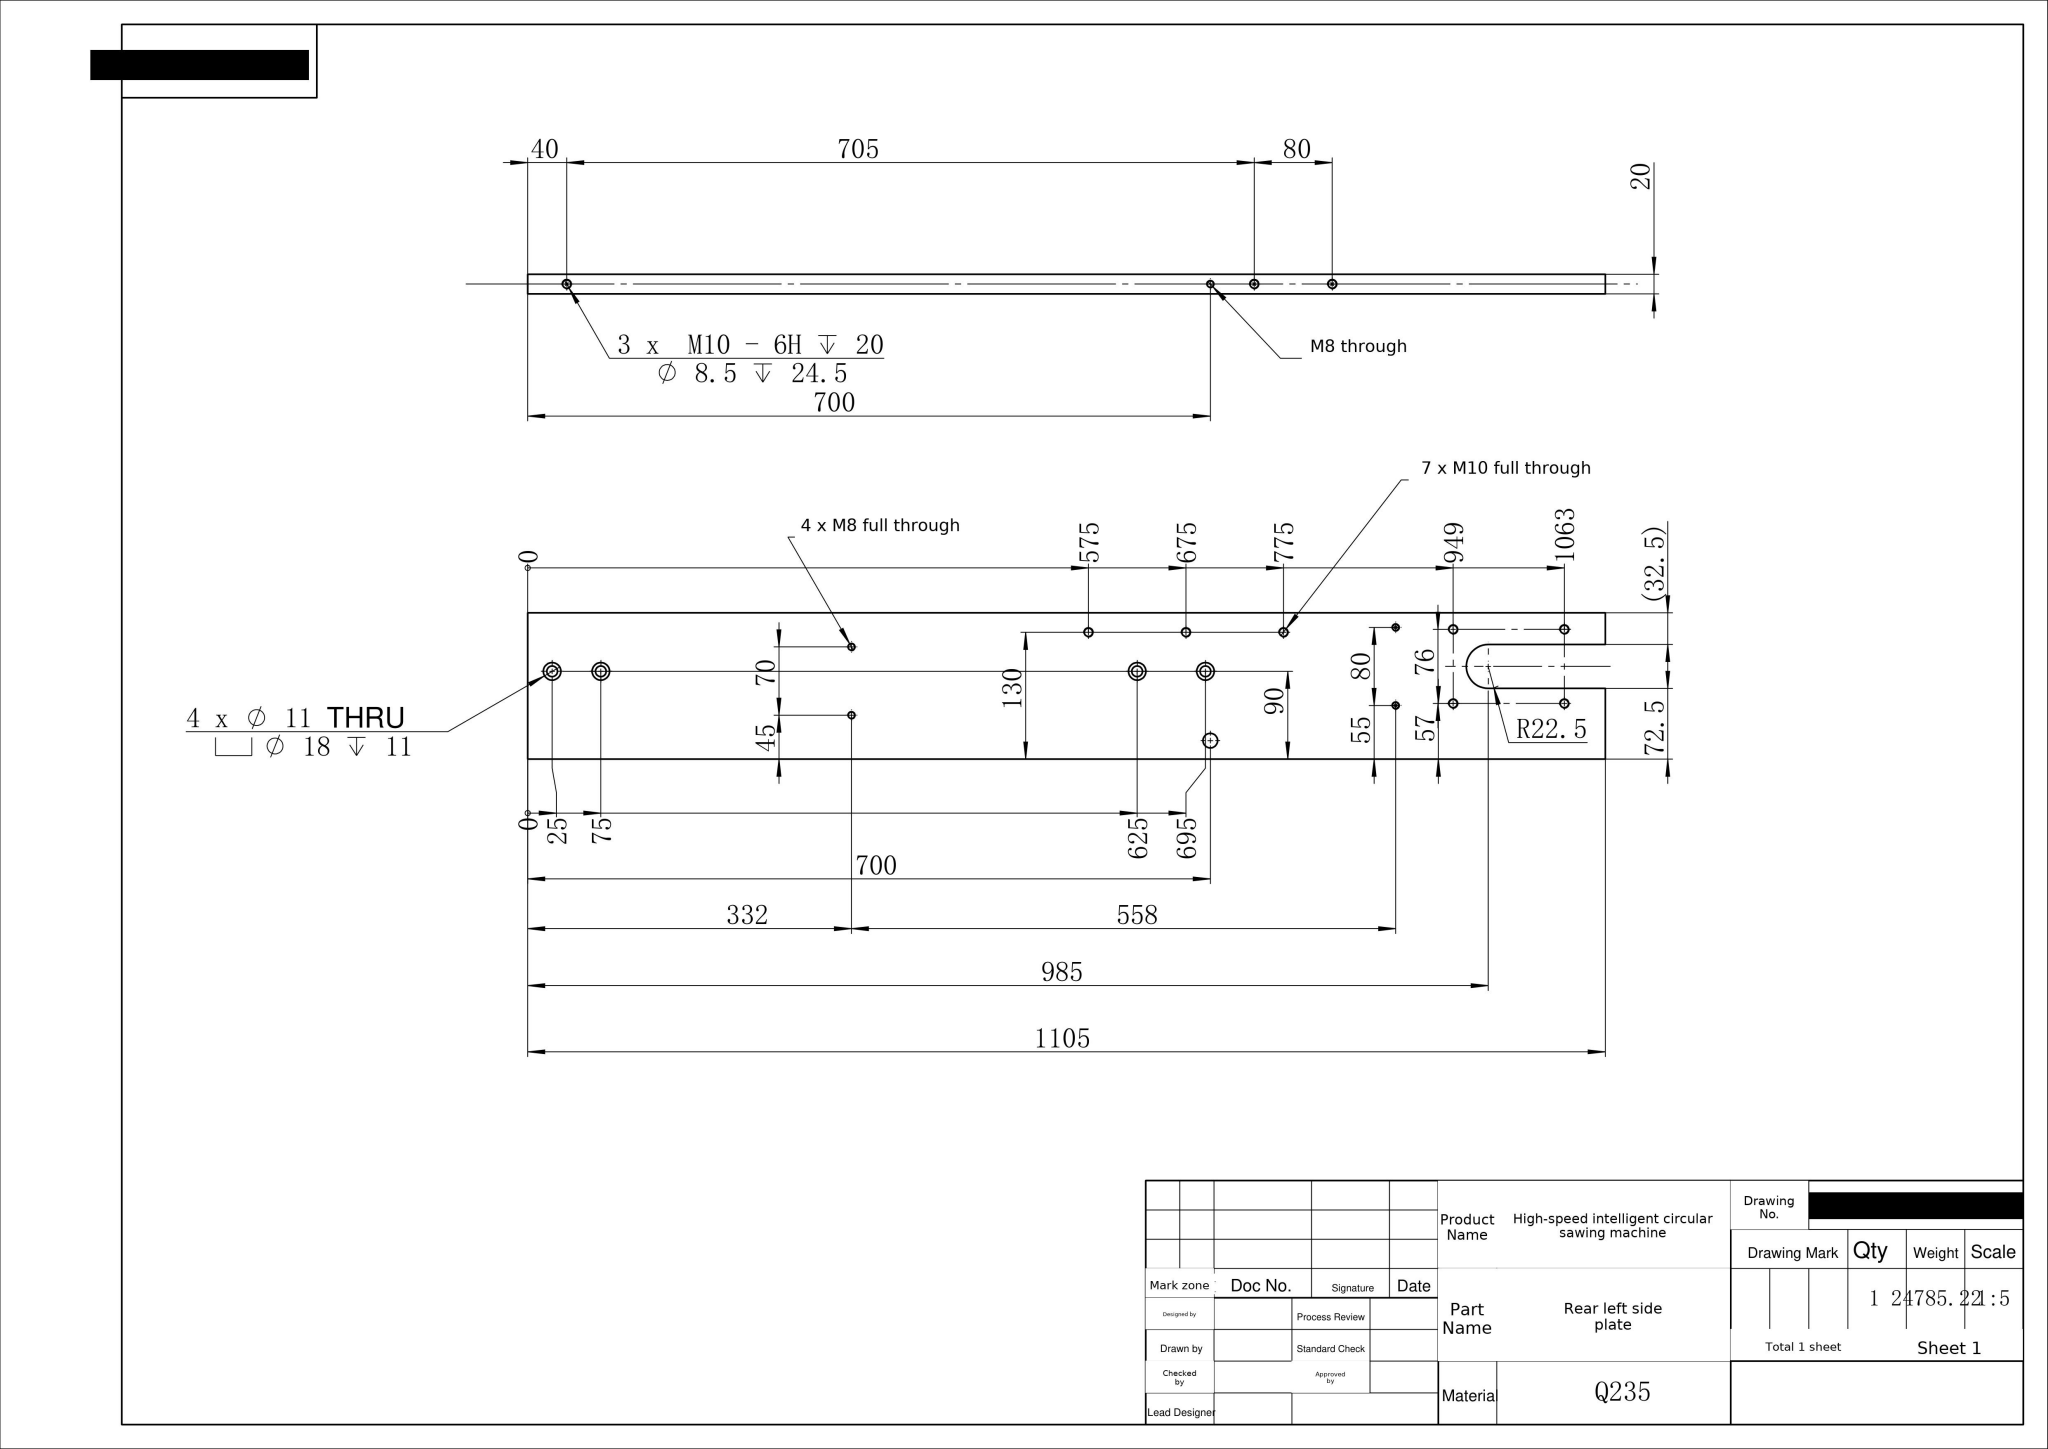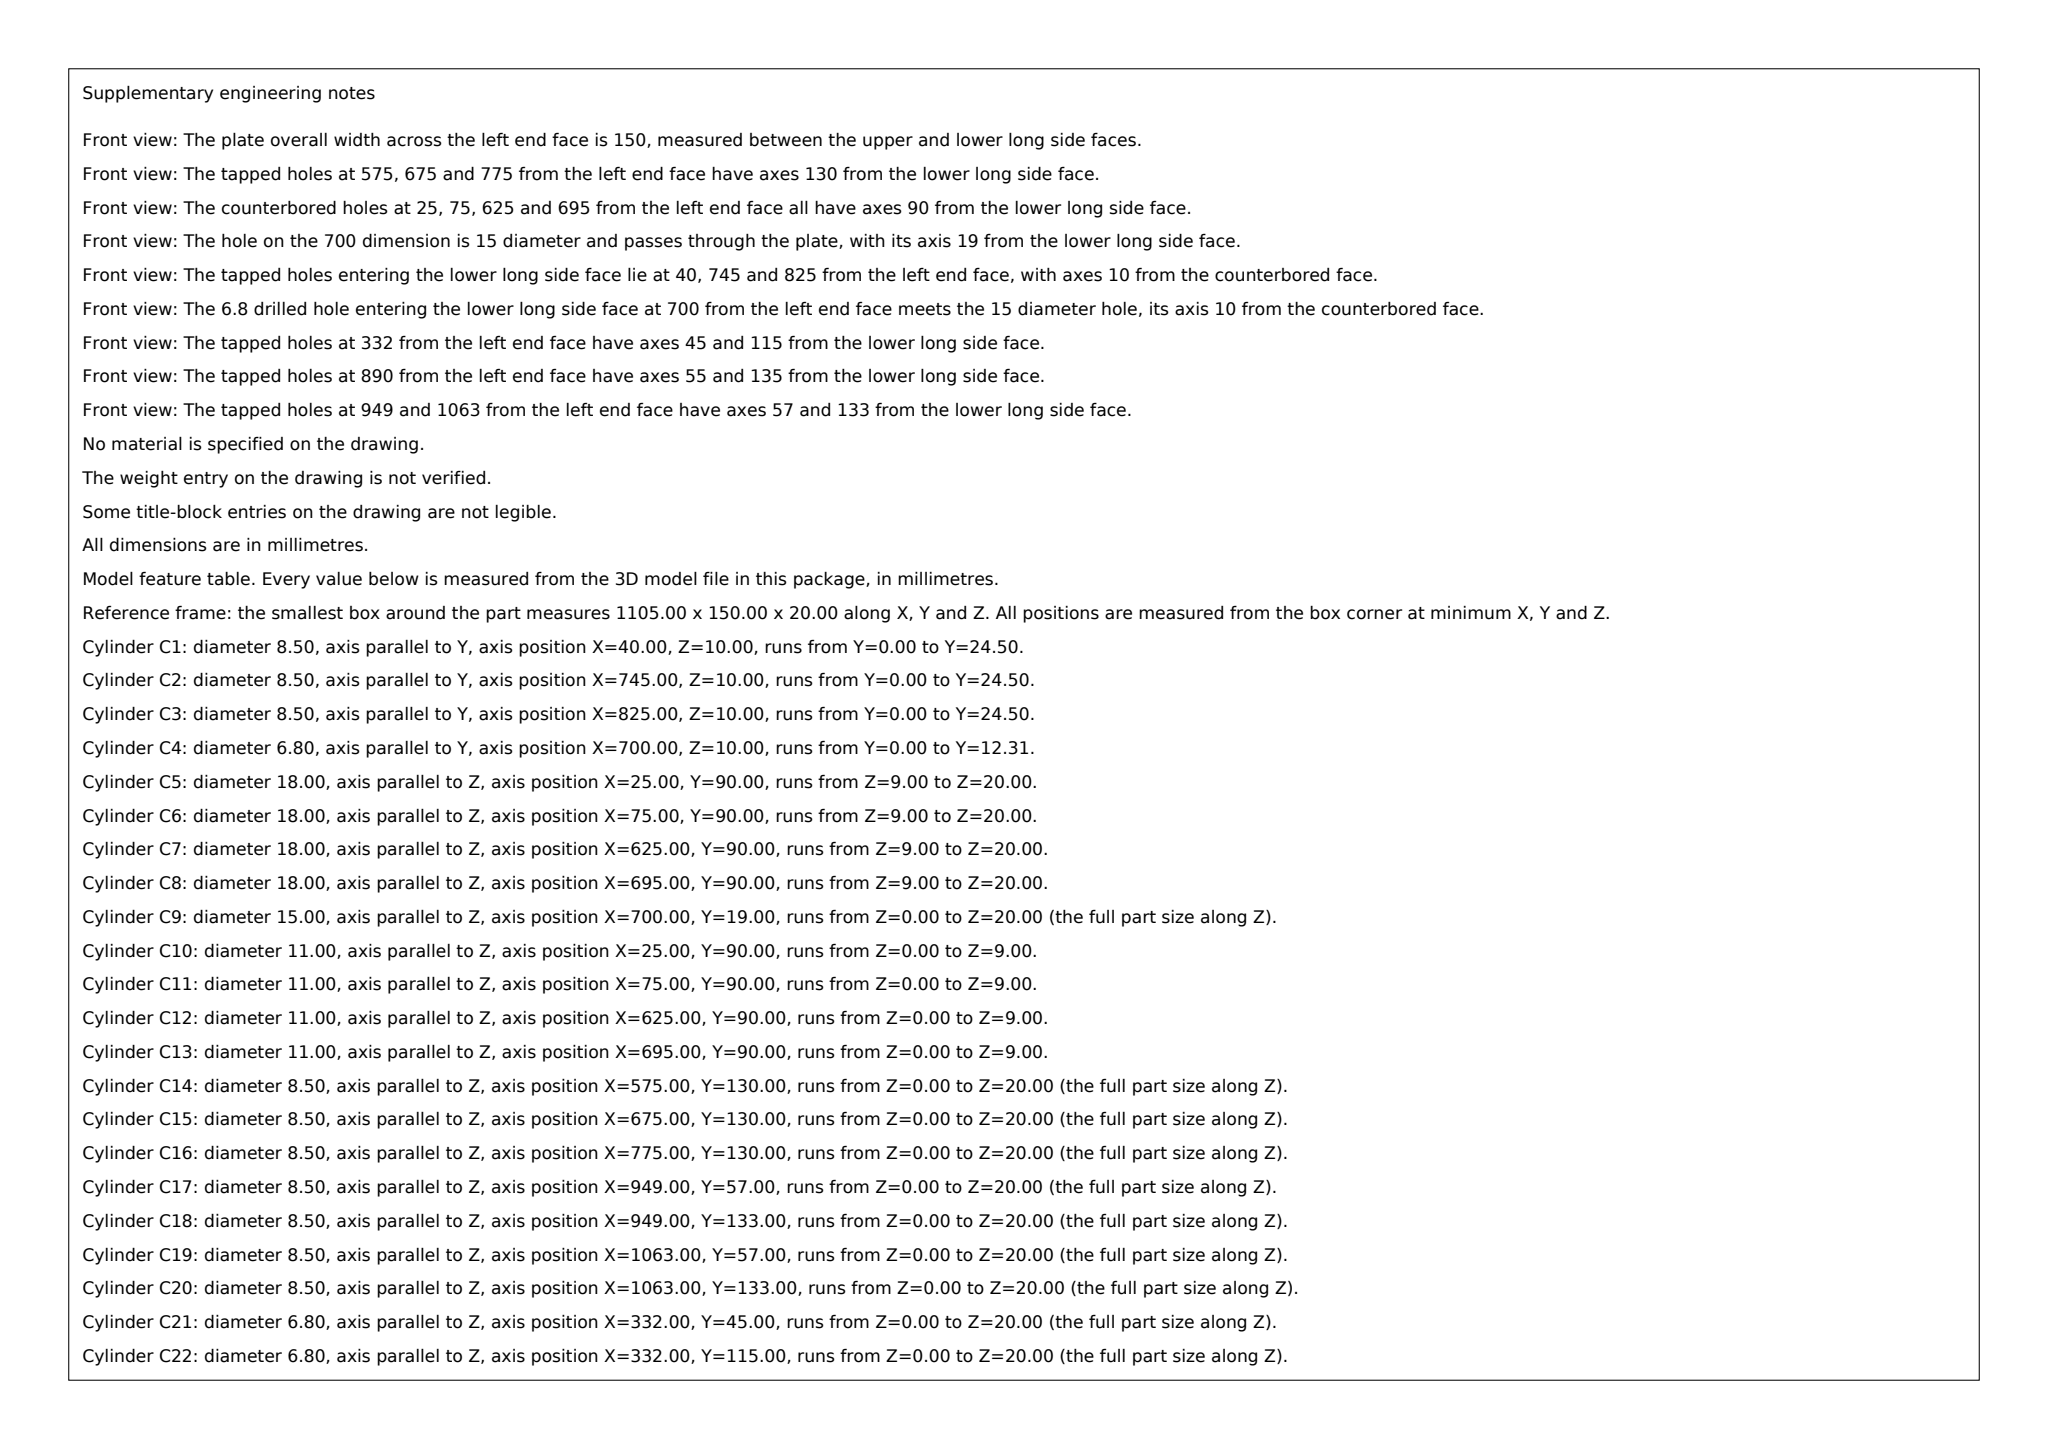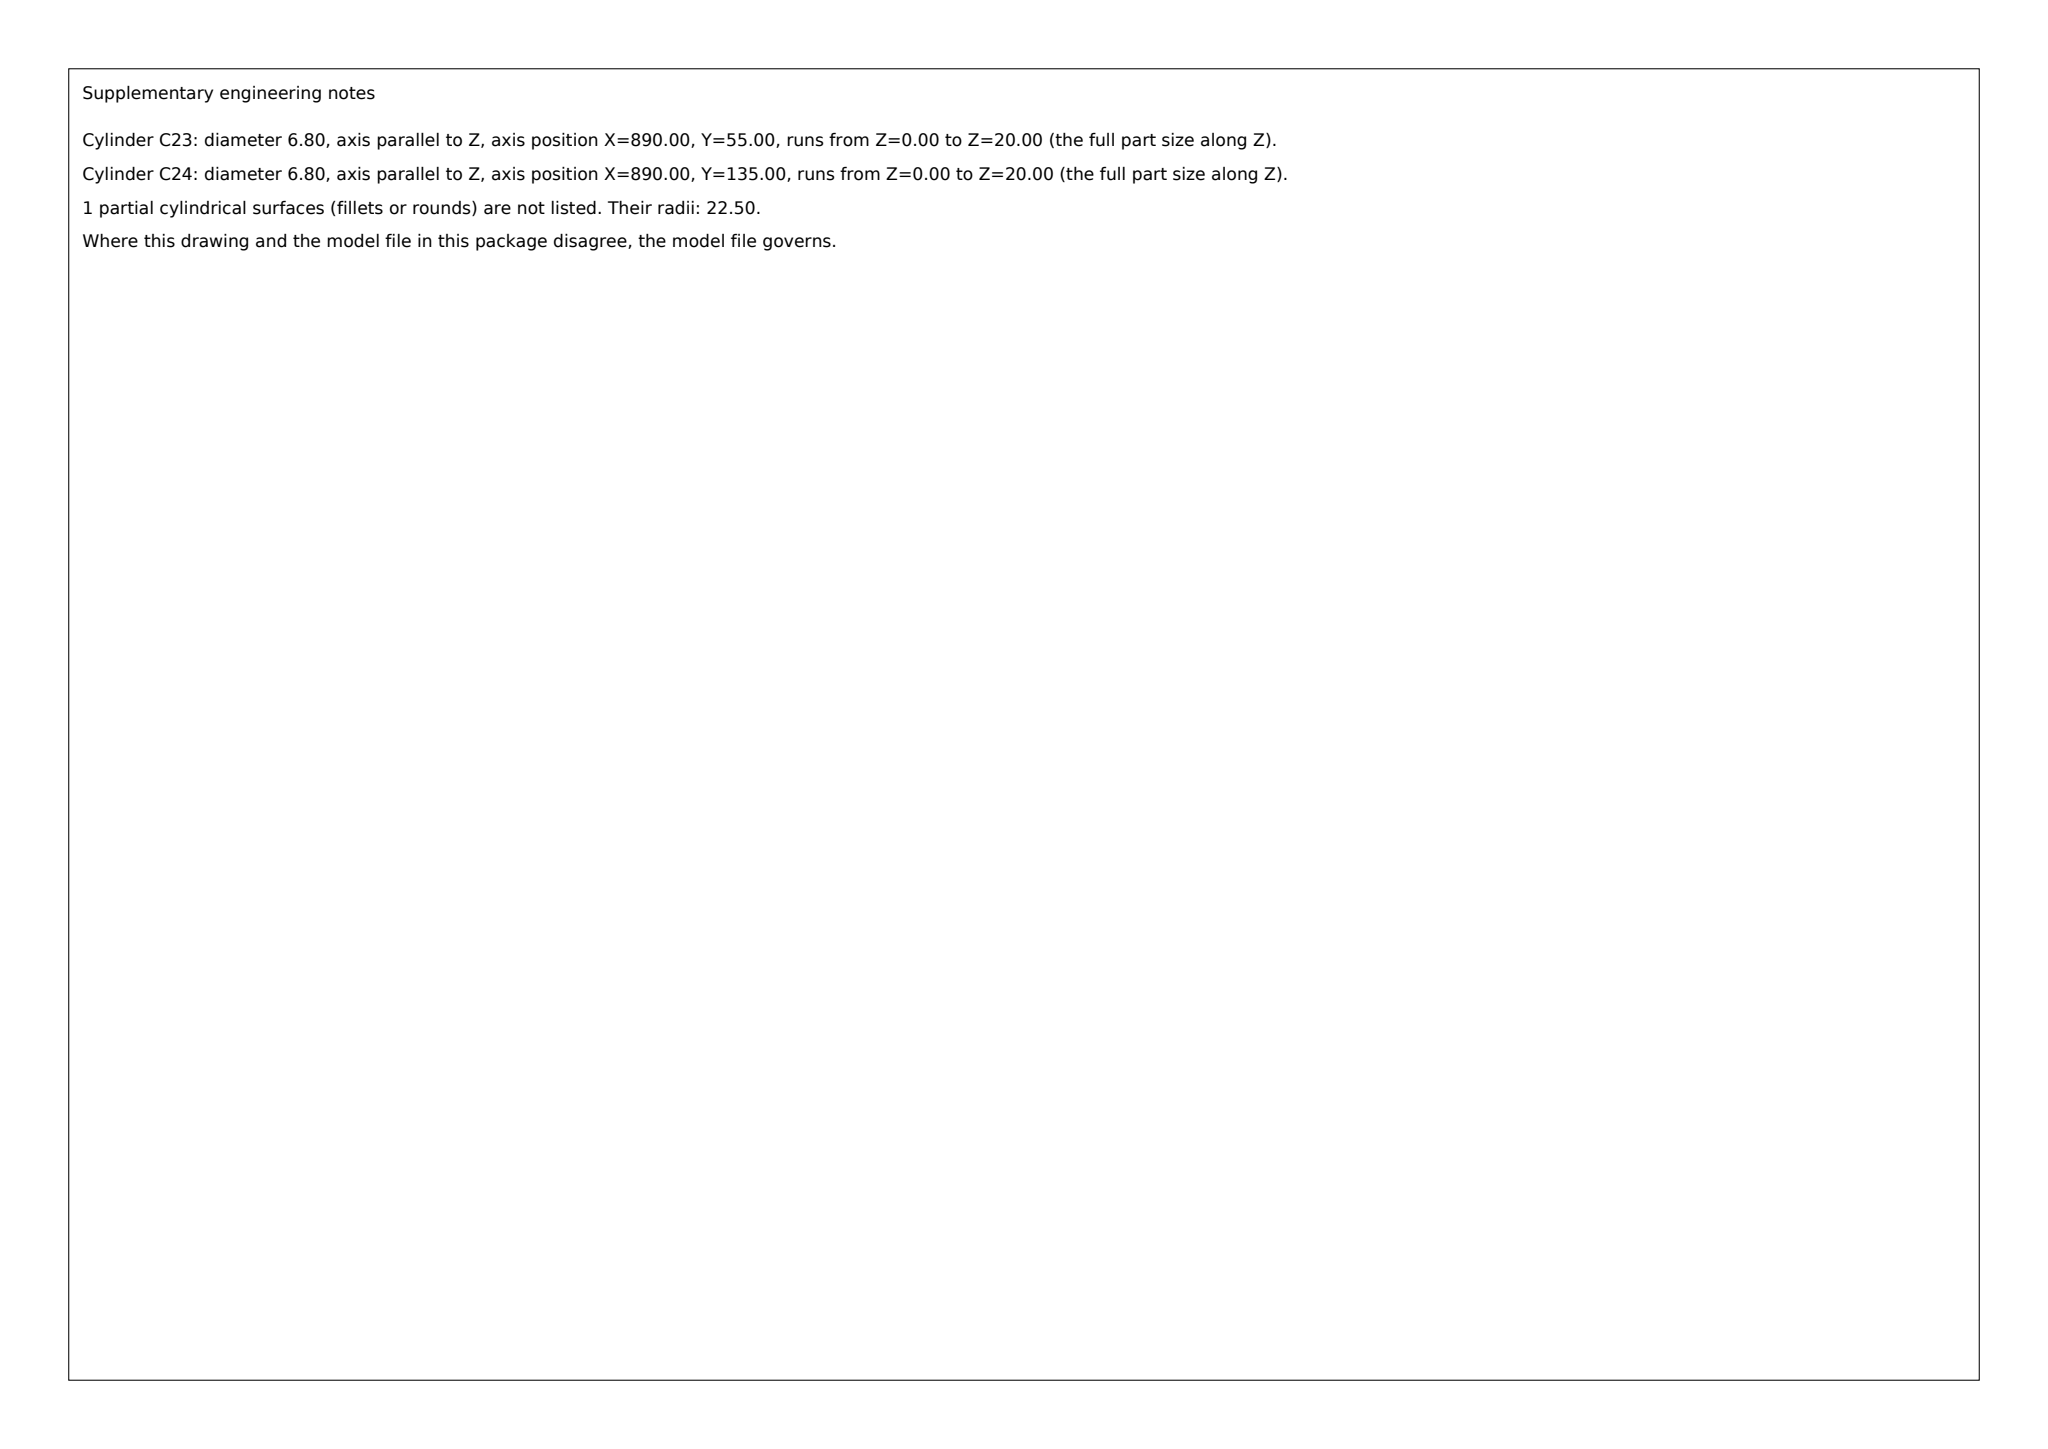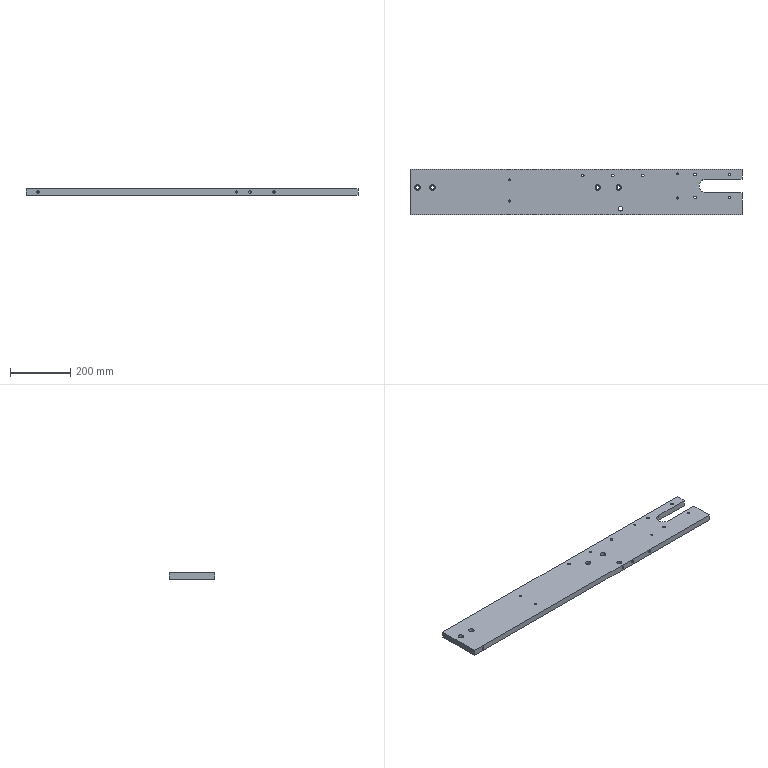Part | SolidWorks | mm | 1 solid | 68 faces | box 1105 x 150 x 20 mm | volume 3157353 mm3 | cylinder 49 | plane 13 | cone 6 | commonest cylinder face diameters 8.5 x20 6.8 x10 18 x8 11 x8 15 x2 45 x1
Drawing notes:
1X Ø15 THRU (20 THK), located X=700, Y=19 from lower-left corner of plate | from the solid: cylinder dia 15.0, axis z, pos [700.0, 19.0], length 20.0 = plate thickness (z planes at 0.0 and 20.0)
UNLESS OTHERWISE SPECIFIED, ALL DIMENSIONS ARE IN MILLIMETERS | from the solid: STEP model facts stated in mm
build123d program:
from build123d import *

# Parameters (mm, degrees)
SKETCH3_R                                          = 31
BOSS_EXTRUDE1_DEPTH                                = 20
HOLE_SIZE_ACCORDING_TO_TYPE_1_OF_HEXAG_D           = 11
HOLE_SIZE_ACCORDING_TO_TYPE_1_OF_HEXAG_CBORE_D     = 18
HOLE_SIZE_ACCORDING_TO_TYPE_1_OF_HEXAG_CBORE_DEPTH = 11
M8_TAPPED_HOLE1_D                                  = 6.8
SKETCH6_R                                          = 7.5
CUT_EXTRUDE1_DEPTH                                 = 1660.317
M8_TAPPED_HOLE2_REACH                              = 717.961
M8_TAPPED_HOLE2_BORE_R                             = 3.4
M10_TAPPED_HOLE1_D                                 = 8.5
M10_TAPPED_HOLE1_DEPTH                             = 24.5
M10_TAPPED_HOLE1_TIP                               = 2.554
SKETCH11_W                                         = 1105
SKETCH11_H                                         = 150
BOSS_EXTRUDE2_DEPTH                                = 20
HOLE_SIZE_ACCORDING_TO_TYPE_2_OF_H_2_COUNT         = 2
HOLE_SIZE_ACCORDING_TO_TYPE_2_OF_H_2_PITCH         = 50
HOLE_SIZE_ACCORDING_TO_TYPE_2_OF_H_3_COUNT         = 2
HOLE_SIZE_ACCORDING_TO_TYPE_2_OF_H_3_PITCH         = 492.5
HOLE_SIZE_ACCORDING_TO_TYPE_2_OF_H_4_COUNT         = 2
HOLE_SIZE_ACCORDING_TO_TYPE_2_OF_H_4_PITCH         = 562.5
HOLE_SIZE_ACCORDING_TO_TYPE_2_OF_H_5_COUNT         = 2
HOLE_SIZE_ACCORDING_TO_TYPE_2_OF_H_5_PITCH         = 1005
HOLE_SIZE_ACCORDING_TO_TYPE_2_OF_H_6_COUNT         = 2
HOLE_SIZE_ACCORDING_TO_TYPE_2_OF_H_6_PITCH         = 1055
SKETCH13_R                                         = 7.5
CUT_EXTRUDE2_DEPTH                                 = 1660.317
SKETCH15_W                                         = 3.4
SKETCH15_H                                         = 19
M8_TAPPED_HOLE3_AT_2_COUNT                         = 2
M8_TAPPED_HOLE3_AT_2_PITCH                         = 905
BOSS_EXTRUDE3_DEPTH                                = 20
HOLE_SIZE_ACCORDING_TO_TYPE_3_OF_H_2_COUNT         = 2
HOLE_SIZE_ACCORDING_TO_TYPE_3_OF_H_2_PITCH         = 50
HOLE_SIZE_ACCORDING_TO_TYPE_3_OF_H_3_COUNT         = 2
HOLE_SIZE_ACCORDING_TO_TYPE_3_OF_H_3_PITCH         = 670
HOLE_SIZE_ACCORDING_TO_TYPE_3_OF_H_4_COUNT         = 2
HOLE_SIZE_ACCORDING_TO_TYPE_3_OF_H_4_PITCH         = 600
SKETCH18_R                                         = 7.5
CUT_EXTRUDE3_DEPTH                                 = 1660.317
SKETCH20_W                                         = 3.4
SKETCH20_H                                         = 19
SKETCH21_W                                         = 4.25
SKETCH21_H                                         = 20
M10_TAPPED_HOLE2_AT_2_COUNT                        = 2
M10_TAPPED_HOLE2_AT_2_PITCH                        = 76
M10_TAPPED_HOLE2_AT_3_COUNT                        = 2
M10_TAPPED_HOLE2_AT_3_PITCH                        = 137.011
M10_TAPPED_HOLE2_AT_4_COUNT                        = 2
M10_TAPPED_HOLE2_AT_4_PITCH                        = 114
SKETCH23_W                                         = 3.4
SKETCH23_H                                         = 20
M8_TAPPED_HOLE5_AT_2_COUNT                         = 2
M8_TAPPED_HOLE5_AT_2_PITCH                         = 80
M10_TAPPED_HOLE3_AT_2_COUNT                        = 2
M10_TAPPED_HOLE3_AT_2_PITCH                        = 246
M10_TAPPED_HOLE3_AT_3_COUNT                        = 2
M10_TAPPED_HOLE3_AT_3_PITCH                        = 326
M10_TAPPED_HOLE4_AT_2_COUNT                        = 2
M10_TAPPED_HOLE4_AT_2_PITCH                        = 1025
M10_TAPPED_HOLE5_AT_2_COUNT                        = 2
M10_TAPPED_HOLE5_AT_2_PITCH                        = 705
M10_TAPPED_HOLE5_AT_3_COUNT                        = 2
M10_TAPPED_HOLE5_AT_3_PITCH                        = 785
SKETCH33_W                                         = 3.4
SKETCH33_H                                         = 20
M8_TAPPED_HOLE6_AT_2_COUNT                         = 2
M8_TAPPED_HOLE6_AT_2_PITCH                         = 70
SKETCH35_W                                         = 3.4
SKETCH35_H                                         = 20
M8_TAPPED_HOLE7_AT_2_COUNT                         = 2
M8_TAPPED_HOLE7_AT_2_PITCH                         = 70
M8_TAPPED_HOLE7_AT_3_COUNT                         = 2
M8_TAPPED_HOLE7_AT_3_PITCH                         = 500
M8_TAPPED_HOLE7_AT_4_COUNT                         = 2
M8_TAPPED_HOLE7_AT_4_PITCH                         = 504.876
SKETCH37_W                                         = 3.4
SKETCH37_H                                         = 20
M8_TAPPED_HOLE8_AT_2_COUNT                         = 2
M8_TAPPED_HOLE8_AT_2_PITCH                         = 70
SKETCH39_W                                         = 4.25
SKETCH39_H                                         = 20
M10_TAPPED_HOLE6_AT_2_COUNT                        = 2
M10_TAPPED_HOLE6_AT_2_PITCH                        = 305
M10_TAPPED_HOLE6_AT_3_COUNT                        = 2
M10_TAPPED_HOLE6_AT_3_PITCH                        = 610
SKETCH41_W                                         = 4.25
SKETCH41_H                                         = 20
M10_TAPPED_HOLE7_AT_2_COUNT                        = 2
M10_TAPPED_HOLE7_AT_2_PITCH                        = 100
M10_TAPPED_HOLE7_AT_3_COUNT                        = 2
M10_TAPPED_HOLE7_AT_3_PITCH                        = 200
SKETCH42_W                                         = 2254.677
SKETCH42_H                                         = 350.493
CUT_EXTRUDE4_DEPTH                                 = 1660.317


with BuildPart() as part:
    # Sketch3 → Boss-Extrude1 (new body)
    with BuildSketch(Plane.XY):
        Polygon((-552.5, 75), (-552.5, -75), (-1657.5, -75), (-1657.5, 50), (-1614.199, 75), align=None)
        with Locations((-1582.5, 20)):
            Circle(SKETCH3_R, mode=Mode.SUBTRACT)
    extrude(amount=-BOSS_EXTRUDE1_DEPTH)

    # Hole Size _according to_ Type 1 of Hexag (through all)
    with Locations(Plane(origin=(-1297.5, 15, 0), x_dir=(1, 0, 0), z_dir=(0, 0, 1))):
        with Locations((0, 0), (70, 0), (670, 0), (720, 0)):
            CounterBoreHole(HOLE_SIZE_ACCORDING_TO_TYPE_1_OF_HEXAG_D / 2, HOLE_SIZE_ACCORDING_TO_TYPE_1_OF_HEXAG_CBORE_D / 2, HOLE_SIZE_ACCORDING_TO_TYPE_1_OF_HEXAG_CBORE_DEPTH)

    # M8 Tapped Hole1 (through all)
    with Locations(Plane(origin=(-1620.5, 20, 0), x_dir=(1, 0, 0), z_dir=(0, 0, 1))):
        with Locations((0, 0), (38, -38), (76, 0), (38, 38)):
            Hole(M8_TAPPED_HOLE1_D / 2)

    # Sketch6 → Cut-Extrude1 (cut, through all)
    with BuildSketch(Plane.XY):
        with Locations((-1252.5, -56)):
            Circle(SKETCH6_R)
    extrude(amount=-CUT_EXTRUDE1_DEPTH, mode=Mode.SUBTRACT)

    # M8 Tapped Hole2 bore (on position points) → M8 Tapped Hole2 (cut, up to next)
    with BuildSketch(Plane(origin=(-1252.5, -75, -10), x_dir=(0, 0, -1), z_dir=(0, -1, 0)), mode=Mode.PRIVATE) as m8_tapped_hole2_sk1:
        Circle(M8_TAPPED_HOLE2_BORE_R)
    m8_tapped_hole2_tool1 = extrude(m8_tapped_hole2_sk1.sketch, amount=-M8_TAPPED_HOLE2_REACH, mode=Mode.PRIVATE) & part.part
    add(m8_tapped_hole2_tool1.solids().sort_by_distance((-1252.5, -75, -10))[0], mode=Mode.SUBTRACT)

    # M10 Tapped Hole1
    with Locations(Plane(origin=(-1657.5, -5, -10), x_dir=(0, 0, -1), z_dir=(-1, 0, 0))):
        with Locations((0, 0), (0, 50)):
            Hole(M10_TAPPED_HOLE1_D / 2, depth=M10_TAPPED_HOLE1_DEPTH)
            with Locations((0, 0, -(M10_TAPPED_HOLE1_DEPTH + M10_TAPPED_HOLE1_TIP / 2))):  # 118° drill point
                Cone(0, M10_TAPPED_HOLE1_D / 2, M10_TAPPED_HOLE1_TIP, mode=Mode.SUBTRACT)

    # Sketch25 → M10 Tapped Hole3 (revolve, cut)
    with BuildSketch(Plane(origin=(-592.5, -75, -10), x_dir=(0, 0, -1), z_dir=(1, 0, 0))):
        Polygon((0, 0), (0, 27.054), (4.25, 24.5), (4.25, 0), align=None)
    m10_tapped_hole3 = revolve(axis=Axis((-592.5, -81.35, -10), (0, 1, 0)), mode=Mode.SUBTRACT)

    # M10 Tapped Hole3 at 2: M10 Tapped Hole3 ×2
    with Locations(*[(-i * M10_TAPPED_HOLE3_AT_2_PITCH, 0, 0) for i in range(1, M10_TAPPED_HOLE3_AT_2_COUNT)]):
        add(m10_tapped_hole3, mode=Mode.SUBTRACT)

    # M10 Tapped Hole3 at 3: M10 Tapped Hole3 ×2
    with Locations(*[(-i * M10_TAPPED_HOLE3_AT_3_PITCH, 0, 0) for i in range(1, M10_TAPPED_HOLE3_AT_3_COUNT)]):
        add(m10_tapped_hole3, mode=Mode.SUBTRACT)

    # Sketch33 → M8 Tapped Hole6 (revolve, cut)
    with BuildSketch(Plane(origin=(-595.5, 40, 0), x_dir=(0, -1, 0), z_dir=(1, 0, 0))):
        with Locations((1.7, 10)):
            Rectangle(SKETCH33_W, SKETCH33_H)
    m8_tapped_hole6 = revolve(axis=Axis((-595.5, 40, 6.35), (0, 0, -1)), mode=Mode.SUBTRACT)

    # M8 Tapped Hole6 at 2: M8 Tapped Hole6 ×2
    with Locations(*[(0, -i * M8_TAPPED_HOLE6_AT_2_PITCH, 0) for i in range(1, M8_TAPPED_HOLE6_AT_2_COUNT)]):
        add(m8_tapped_hole6, mode=Mode.SUBTRACT)

    # Sketch39 → M10 Tapped Hole6 (revolve, cut)
    with BuildSketch(Plane(origin=(-1511.5, 55, 0), x_dir=(0, -1, 0), z_dir=(1, 0, 0))):
        with Locations((2.125, 10)):
            Rectangle(SKETCH39_W, SKETCH39_H)
    m10_tapped_hole6 = revolve(axis=Axis((-1511.5, 55, 6.35), (0, 0, -1)), mode=Mode.SUBTRACT)

    # M10 Tapped Hole6 at 2: M10 Tapped Hole6 ×2
    with Locations(*[(i * M10_TAPPED_HOLE6_AT_2_PITCH, 0, 0) for i in range(1, M10_TAPPED_HOLE6_AT_2_COUNT)]):
        add(m10_tapped_hole6, mode=Mode.SUBTRACT)

    # M10 Tapped Hole6 at 3: M10 Tapped Hole6 ×2
    with Locations(*[(i * M10_TAPPED_HOLE6_AT_3_PITCH, 0, 0) for i in range(1, M10_TAPPED_HOLE6_AT_3_COUNT)]):
        add(m10_tapped_hole6, mode=Mode.SUBTRACT)


with BuildPart() as body_2:
    # Sketch11 → Boss-Extrude2 (new body)
    with BuildSketch(Plane.XY):
        Rectangle(SKETCH11_W, SKETCH11_H)
    extrude(amount=-BOSS_EXTRUDE2_DEPTH)

    # Sketch12 → Hole Size _according to_ Type 2 of Hexag (revolve, cut)
    with BuildSketch(Plane(origin=(-527.5, 15, 0), x_dir=(0, -1, 0), z_dir=(1, 0, 0))):
        Polygon((0, 0), (0, 20), (5.5, 20), (5.5, 11), (9, 11), (9, 0), align=None)
    hole_size_according_to_type_2_of_hexag = revolve(axis=Axis((-527.5, 15, 6.35), (0, 0, -1)), mode=Mode.SUBTRACT)

    # Hole Size _according to_ Type 2 of H 2: Hole Size _according to_ Type 2 of Hexag ×2
    with Locations(*[(i * HOLE_SIZE_ACCORDING_TO_TYPE_2_OF_H_2_PITCH, 0, 0) for i in range(1, HOLE_SIZE_ACCORDING_TO_TYPE_2_OF_H_2_COUNT)]):
        add(hole_size_according_to_type_2_of_hexag, mode=Mode.SUBTRACT)

    # Hole Size _according to_ Type 2 of H 3: Hole Size _according to_ Type 2 of Hexag ×2
    with Locations(*[(i * HOLE_SIZE_ACCORDING_TO_TYPE_2_OF_H_3_PITCH, 0, 0) for i in range(1, HOLE_SIZE_ACCORDING_TO_TYPE_2_OF_H_3_COUNT)]):
        add(hole_size_according_to_type_2_of_hexag, mode=Mode.SUBTRACT)

    # Hole Size _according to_ Type 2 of H 4: Hole Size _according to_ Type 2 of Hexag ×2
    with Locations(*[(i * HOLE_SIZE_ACCORDING_TO_TYPE_2_OF_H_4_PITCH, 0, 0) for i in range(1, HOLE_SIZE_ACCORDING_TO_TYPE_2_OF_H_4_COUNT)]):
        add(hole_size_according_to_type_2_of_hexag, mode=Mode.SUBTRACT)

    # Hole Size _according to_ Type 2 of H 5: Hole Size _according to_ Type 2 of Hexag ×2
    with Locations(*[(i * HOLE_SIZE_ACCORDING_TO_TYPE_2_OF_H_5_PITCH, 0, 0) for i in range(1, HOLE_SIZE_ACCORDING_TO_TYPE_2_OF_H_5_COUNT)]):
        add(hole_size_according_to_type_2_of_hexag, mode=Mode.SUBTRACT)

    # Hole Size _according to_ Type 2 of H 6: Hole Size _according to_ Type 2 of Hexag ×2
    with Locations(*[(i * HOLE_SIZE_ACCORDING_TO_TYPE_2_OF_H_6_PITCH, 0, 0) for i in range(1, HOLE_SIZE_ACCORDING_TO_TYPE_2_OF_H_6_COUNT)]):
        add(hole_size_according_to_type_2_of_hexag, mode=Mode.SUBTRACT)

    # Sketch13 → Cut-Extrude2 (cut, through all)
    with BuildSketch(Plane.XY):
        with Locations((452.5, -56)):
            Circle(SKETCH13_R)
        with Locations((-452.5, -56)):
            Circle(SKETCH13_R)
    extrude(amount=-CUT_EXTRUDE2_DEPTH, mode=Mode.SUBTRACT)

    # Sketch15 → M8 Tapped Hole3 (revolve, cut)
    with BuildSketch(Plane(origin=(-452.5, -75, -10), x_dir=(0, 0, -1), z_dir=(1, 0, 0))):
        with Locations((1.7, 9.5)):
            Rectangle(SKETCH15_W, SKETCH15_H)
    m8_tapped_hole3 = revolve(axis=Axis((-452.5, -81.35, -10), (0, 1, 0)), mode=Mode.SUBTRACT)

    # M8 Tapped Hole3 at 2: M8 Tapped Hole3 ×2
    with Locations(*[(i * M8_TAPPED_HOLE3_AT_2_PITCH, 0, 0) for i in range(1, M8_TAPPED_HOLE3_AT_2_COUNT)]):
        add(m8_tapped_hole3, mode=Mode.SUBTRACT)

    # Sketch27 → M10 Tapped Hole4 (revolve, cut)
    with BuildSketch(Plane(origin=(-512.5, -75, -10), x_dir=(0, 0, -1), z_dir=(1, 0, 0))):
        Polygon((0, 0), (0, 27.054), (4.25, 24.5), (4.25, 0), align=None)
    m10_tapped_hole4 = revolve(axis=Axis((-512.5, -81.35, -10), (0, 1, 0)), mode=Mode.SUBTRACT)

    # M10 Tapped Hole4 at 2: M10 Tapped Hole4 ×2
    with Locations(*[(i * M10_TAPPED_HOLE4_AT_2_PITCH, 0, 0) for i in range(1, M10_TAPPED_HOLE4_AT_2_COUNT)]):
        add(m10_tapped_hole4, mode=Mode.SUBTRACT)

    # Sketch35 → M8 Tapped Hole7 (revolve, cut)
    with BuildSketch(Plane(origin=(-105.5, 40, 0), x_dir=(0, -1, 0), z_dir=(1, 0, 0))):
        with Locations((1.7, 10)):
            Rectangle(SKETCH35_W, SKETCH35_H)
    m8_tapped_hole7 = revolve(axis=Axis((-105.5, 40, 6.35), (0, 0, -1)), mode=Mode.SUBTRACT)

    # M8 Tapped Hole7 at 2: M8 Tapped Hole7 ×2
    with Locations(*[(0, -i * M8_TAPPED_HOLE7_AT_2_PITCH, 0) for i in range(1, M8_TAPPED_HOLE7_AT_2_COUNT)]):
        add(m8_tapped_hole7, mode=Mode.SUBTRACT)

    # M8 Tapped Hole7 at 3: M8 Tapped Hole7 ×2
    with Locations(*[(i * M8_TAPPED_HOLE7_AT_3_PITCH, 0, 0) for i in range(1, M8_TAPPED_HOLE7_AT_3_COUNT)]):
        add(m8_tapped_hole7, mode=Mode.SUBTRACT)

    # M8 Tapped Hole7 at 4: M8 Tapped Hole7 ×2
    with Locations(*[Vector(0.9903, -0.1386, 0) * (i * M8_TAPPED_HOLE7_AT_4_PITCH) for i in range(1, M8_TAPPED_HOLE7_AT_4_COUNT)]):
        add(m8_tapped_hole7, mode=Mode.SUBTRACT)


with BuildPart() as body_3:
    # Sketch16 → Boss-Extrude3 (new body)
    with BuildSketch(Plane.XY):
        with BuildLine():
            Line((552.5, 75), (1657.5, 75))
            Line((1657.5, 75), (1657.5, 42.5))
            Line((1657.5, 42.5), (1537.5, 42.5))
            ThreePointArc((1537.5, 42.5), (1515, 20), (1537.5, -2.5))
            Line((1537.5, -2.5), (1657.5, -2.5))
            Line((1657.5, -2.5), (1657.5, -75))
            Line((1657.5, -75), (552.5, -75))
            Line((552.5, -75), (552.5, 75))
        make_face()
    extrude(amount=-BOSS_EXTRUDE3_DEPTH)

    # Sketch17 → Hole Size _according to_ Type 3 of Hexag (revolve, cut)
    with BuildSketch(Plane(origin=(577.5, 15, 0), x_dir=(0, -1, 0), z_dir=(1, 0, 0))):
        Polygon((0, 0), (0, 20), (5.5, 20), (5.5, 11), (9, 11), (9, 0), align=None)
    hole_size_according_to_type_3_of_hexag = revolve(axis=Axis((577.5, 15, 6.35), (0, 0, -1)), mode=Mode.SUBTRACT)

    # Hole Size _according to_ Type 3 of H 2: Hole Size _according to_ Type 3 of Hexag ×2
    with Locations(*[(i * HOLE_SIZE_ACCORDING_TO_TYPE_3_OF_H_2_PITCH, 0, 0) for i in range(1, HOLE_SIZE_ACCORDING_TO_TYPE_3_OF_H_2_COUNT)]):
        add(hole_size_according_to_type_3_of_hexag, mode=Mode.SUBTRACT)

    # Hole Size _according to_ Type 3 of H 3: Hole Size _according to_ Type 3 of Hexag ×2
    with Locations(*[(i * HOLE_SIZE_ACCORDING_TO_TYPE_3_OF_H_3_PITCH, 0, 0) for i in range(1, HOLE_SIZE_ACCORDING_TO_TYPE_3_OF_H_3_COUNT)]):
        add(hole_size_according_to_type_3_of_hexag, mode=Mode.SUBTRACT)

    # Hole Size _according to_ Type 3 of H 4: Hole Size _according to_ Type 3 of Hexag ×2
    with Locations(*[(i * HOLE_SIZE_ACCORDING_TO_TYPE_3_OF_H_4_PITCH, 0, 0) for i in range(1, HOLE_SIZE_ACCORDING_TO_TYPE_3_OF_H_4_COUNT)]):
        add(hole_size_according_to_type_3_of_hexag, mode=Mode.SUBTRACT)

    # Sketch18 → Cut-Extrude3 (cut, through all)
    with BuildSketch(Plane.XY):
        with Locations((1252.5, -56)):
            Circle(SKETCH18_R)
    extrude(amount=-CUT_EXTRUDE3_DEPTH, mode=Mode.SUBTRACT)

    # Sketch20 → M8 Tapped Hole4 (revolve, cut)
    with BuildSketch(Plane(origin=(1252.5, -75, -10), x_dir=(0, 0, -1), z_dir=(1, 0, 0))):
        with Locations((1.7, 9.5)):
            Rectangle(SKETCH20_W, SKETCH20_H)
    revolve(axis=Axis((1252.5, -81.35, -10), (0, 1, 0)), mode=Mode.SUBTRACT)

    # Sketch21 → M10 Tapped Hole2 (revolve, cut)
    with BuildSketch(Plane(origin=(1501.5, 58, 0), x_dir=(0, -1, 0), z_dir=(1, 0, 0))):
        with Locations((2.125, 10)):
            Rectangle(SKETCH21_W, SKETCH21_H)
    m10_tapped_hole2 = revolve(axis=Axis((1501.5, 58, 6.35), (0, 0, -1)), mode=Mode.SUBTRACT)

    # M10 Tapped Hole2 at 2: M10 Tapped Hole2 ×2
    with Locations(*[(0, -i * M10_TAPPED_HOLE2_AT_2_PITCH, 0) for i in range(1, M10_TAPPED_HOLE2_AT_2_COUNT)]):
        add(m10_tapped_hole2, mode=Mode.SUBTRACT)

    # M10 Tapped Hole2 at 3: M10 Tapped Hole2 ×2
    with Locations(*[Vector(0.8321, -0.5547, 0) * (i * M10_TAPPED_HOLE2_AT_3_PITCH) for i in range(1, M10_TAPPED_HOLE2_AT_3_COUNT)]):
        add(m10_tapped_hole2, mode=Mode.SUBTRACT)

    # M10 Tapped Hole2 at 4: M10 Tapped Hole2 ×2
    with Locations(*[(i * M10_TAPPED_HOLE2_AT_4_PITCH, 0, 0) for i in range(1, M10_TAPPED_HOLE2_AT_4_COUNT)]):
        add(m10_tapped_hole2, mode=Mode.SUBTRACT)

    # Sketch23 → M8 Tapped Hole5 (revolve, cut)
    with BuildSketch(Plane(origin=(1442.5, 60, 0), x_dir=(0, -1, 0), z_dir=(1, 0, 0))):
        with Locations((1.7, 10)):
            Rectangle(SKETCH23_W, SKETCH23_H)
    m8_tapped_hole5 = revolve(axis=Axis((1442.5, 60, 6.35), (0, 0, -1)), mode=Mode.SUBTRACT)

    # M8 Tapped Hole5 at 2: M8 Tapped Hole5 ×2
    with Locations(*[(0, -i * M8_TAPPED_HOLE5_AT_2_PITCH, 0) for i in range(1, M8_TAPPED_HOLE5_AT_2_COUNT)]):
        add(m8_tapped_hole5, mode=Mode.SUBTRACT)

    # Sketch31 → M10 Tapped Hole5 (revolve, cut)
    with BuildSketch(Plane(origin=(592.5, -75, -10), x_dir=(0, 0, -1), z_dir=(1, 0, 0))):
        Polygon((0, 0), (0, 27.054), (4.25, 24.5), (4.25, 0), align=None)
    m10_tapped_hole5 = revolve(axis=Axis((592.5, -81.35, -10), (0, 1, 0)), mode=Mode.SUBTRACT)

    # M10 Tapped Hole5 at 2: M10 Tapped Hole5 ×2
    with Locations(*[(i * M10_TAPPED_HOLE5_AT_2_PITCH, 0, 0) for i in range(1, M10_TAPPED_HOLE5_AT_2_COUNT)]):
        add(m10_tapped_hole5, mode=Mode.SUBTRACT)

    # M10 Tapped Hole5 at 3: M10 Tapped Hole5 ×2
    with Locations(*[(i * M10_TAPPED_HOLE5_AT_3_PITCH, 0, 0) for i in range(1, M10_TAPPED_HOLE5_AT_3_COUNT)]):
        add(m10_tapped_hole5, mode=Mode.SUBTRACT)

    # Sketch37 → M8 Tapped Hole8 (revolve, cut)
    with BuildSketch(Plane(origin=(884.5, 40, 0), x_dir=(0, -1, 0), z_dir=(1, 0, 0))):
        with Locations((1.7, 10)):
            Rectangle(SKETCH37_W, SKETCH37_H)
    m8_tapped_hole8 = revolve(axis=Axis((884.5, 40, 6.35), (0, 0, -1)), mode=Mode.SUBTRACT)

    # M8 Tapped Hole8 at 2: M8 Tapped Hole8 ×2
    with Locations(*[(0, -i * M8_TAPPED_HOLE8_AT_2_PITCH, 0) for i in range(1, M8_TAPPED_HOLE8_AT_2_COUNT)]):
        add(m8_tapped_hole8, mode=Mode.SUBTRACT)

    # Sketch41 → M10 Tapped Hole7 (revolve, cut)
    with BuildSketch(Plane(origin=(1127.5, 55, 0), x_dir=(0, -1, 0), z_dir=(1, 0, 0))):
        with Locations((2.125, 10)):
            Rectangle(SKETCH41_W, SKETCH41_H)
    m10_tapped_hole7 = revolve(axis=Axis((1127.5, 55, 6.35), (0, 0, -1)), mode=Mode.SUBTRACT)

    # M10 Tapped Hole7 at 2: M10 Tapped Hole7 ×2
    with Locations(*[(i * M10_TAPPED_HOLE7_AT_2_PITCH, 0, 0) for i in range(1, M10_TAPPED_HOLE7_AT_2_COUNT)]):
        add(m10_tapped_hole7, mode=Mode.SUBTRACT)

    # M10 Tapped Hole7 at 3: M10 Tapped Hole7 ×2
    with Locations(*[(i * M10_TAPPED_HOLE7_AT_3_PITCH, 0, 0) for i in range(1, M10_TAPPED_HOLE7_AT_3_COUNT)]):
        add(m10_tapped_hole7, mode=Mode.SUBTRACT)


with BuildPart() as cut_extrude4_tool:
    # Sketch42 → Cut-Extrude4 (new, through all)
    with BuildSketch(Plane(origin=(0, 0, -20), x_dir=(-1, 0, 0), z_dir=(0, 0, -1))):
        with Locations((574.838, -100.247)):
            Rectangle(SKETCH42_W, SKETCH42_H)
    extrude(amount=-CUT_EXTRUDE4_DEPTH)


with BuildPart() as part_1:
    add(part.part)

    # Cut-Extrude4: cut by cut_extrude4_tool
    add(cut_extrude4_tool.part, mode=Mode.SUBTRACT)


with BuildPart() as body_2_1:
    add(body_2.part)

    # Cut-Extrude4: cut by cut_extrude4_tool
    add(cut_extrude4_tool.part, mode=Mode.SUBTRACT)


solid = body_3.part